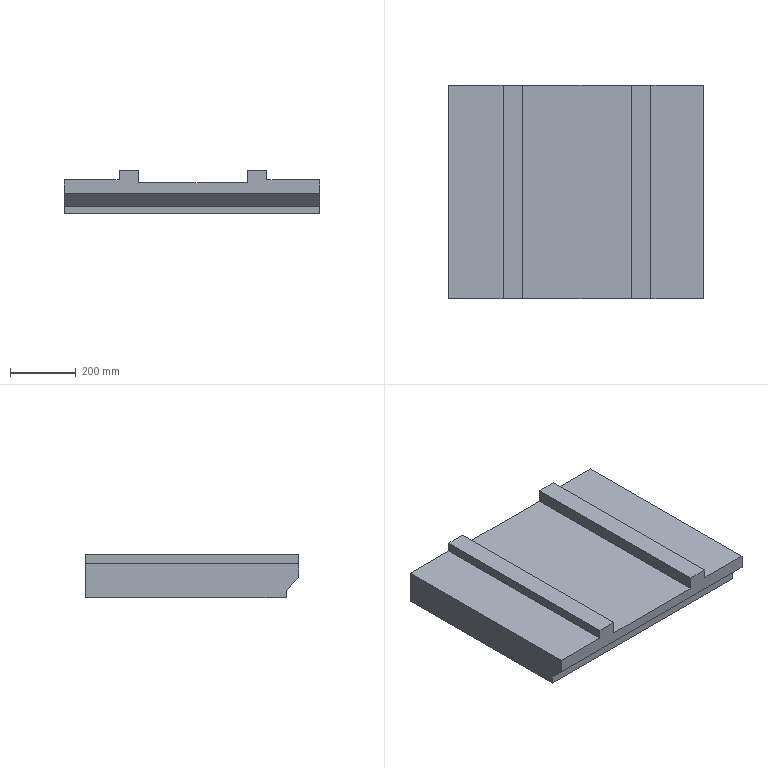Component | NX | SIM15_Z1_SCHLITTEN | 1 solid | 16 faces | volume 51708230 mm3 | plane 16